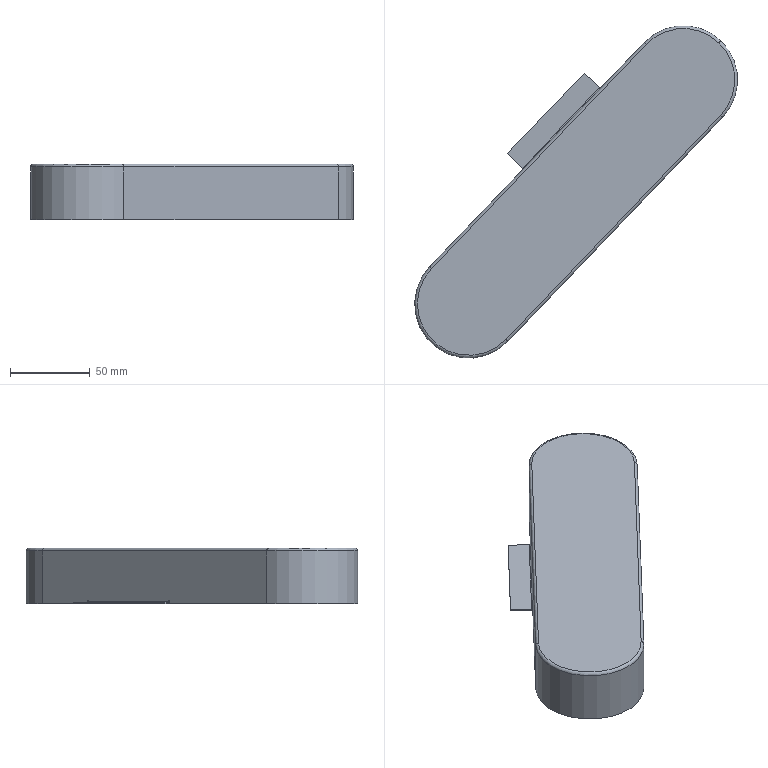Component | SolidWorks | LD101-02--Q1071-Q1-2-1 | 1 solid | 42 faces | volume 37929 mm3 | plane 24 | cylinder 12 | torus 6 | commonest cylinder face diameters 66 x3 68 x3 3.473 x3 1.473 x3 | material SUS304